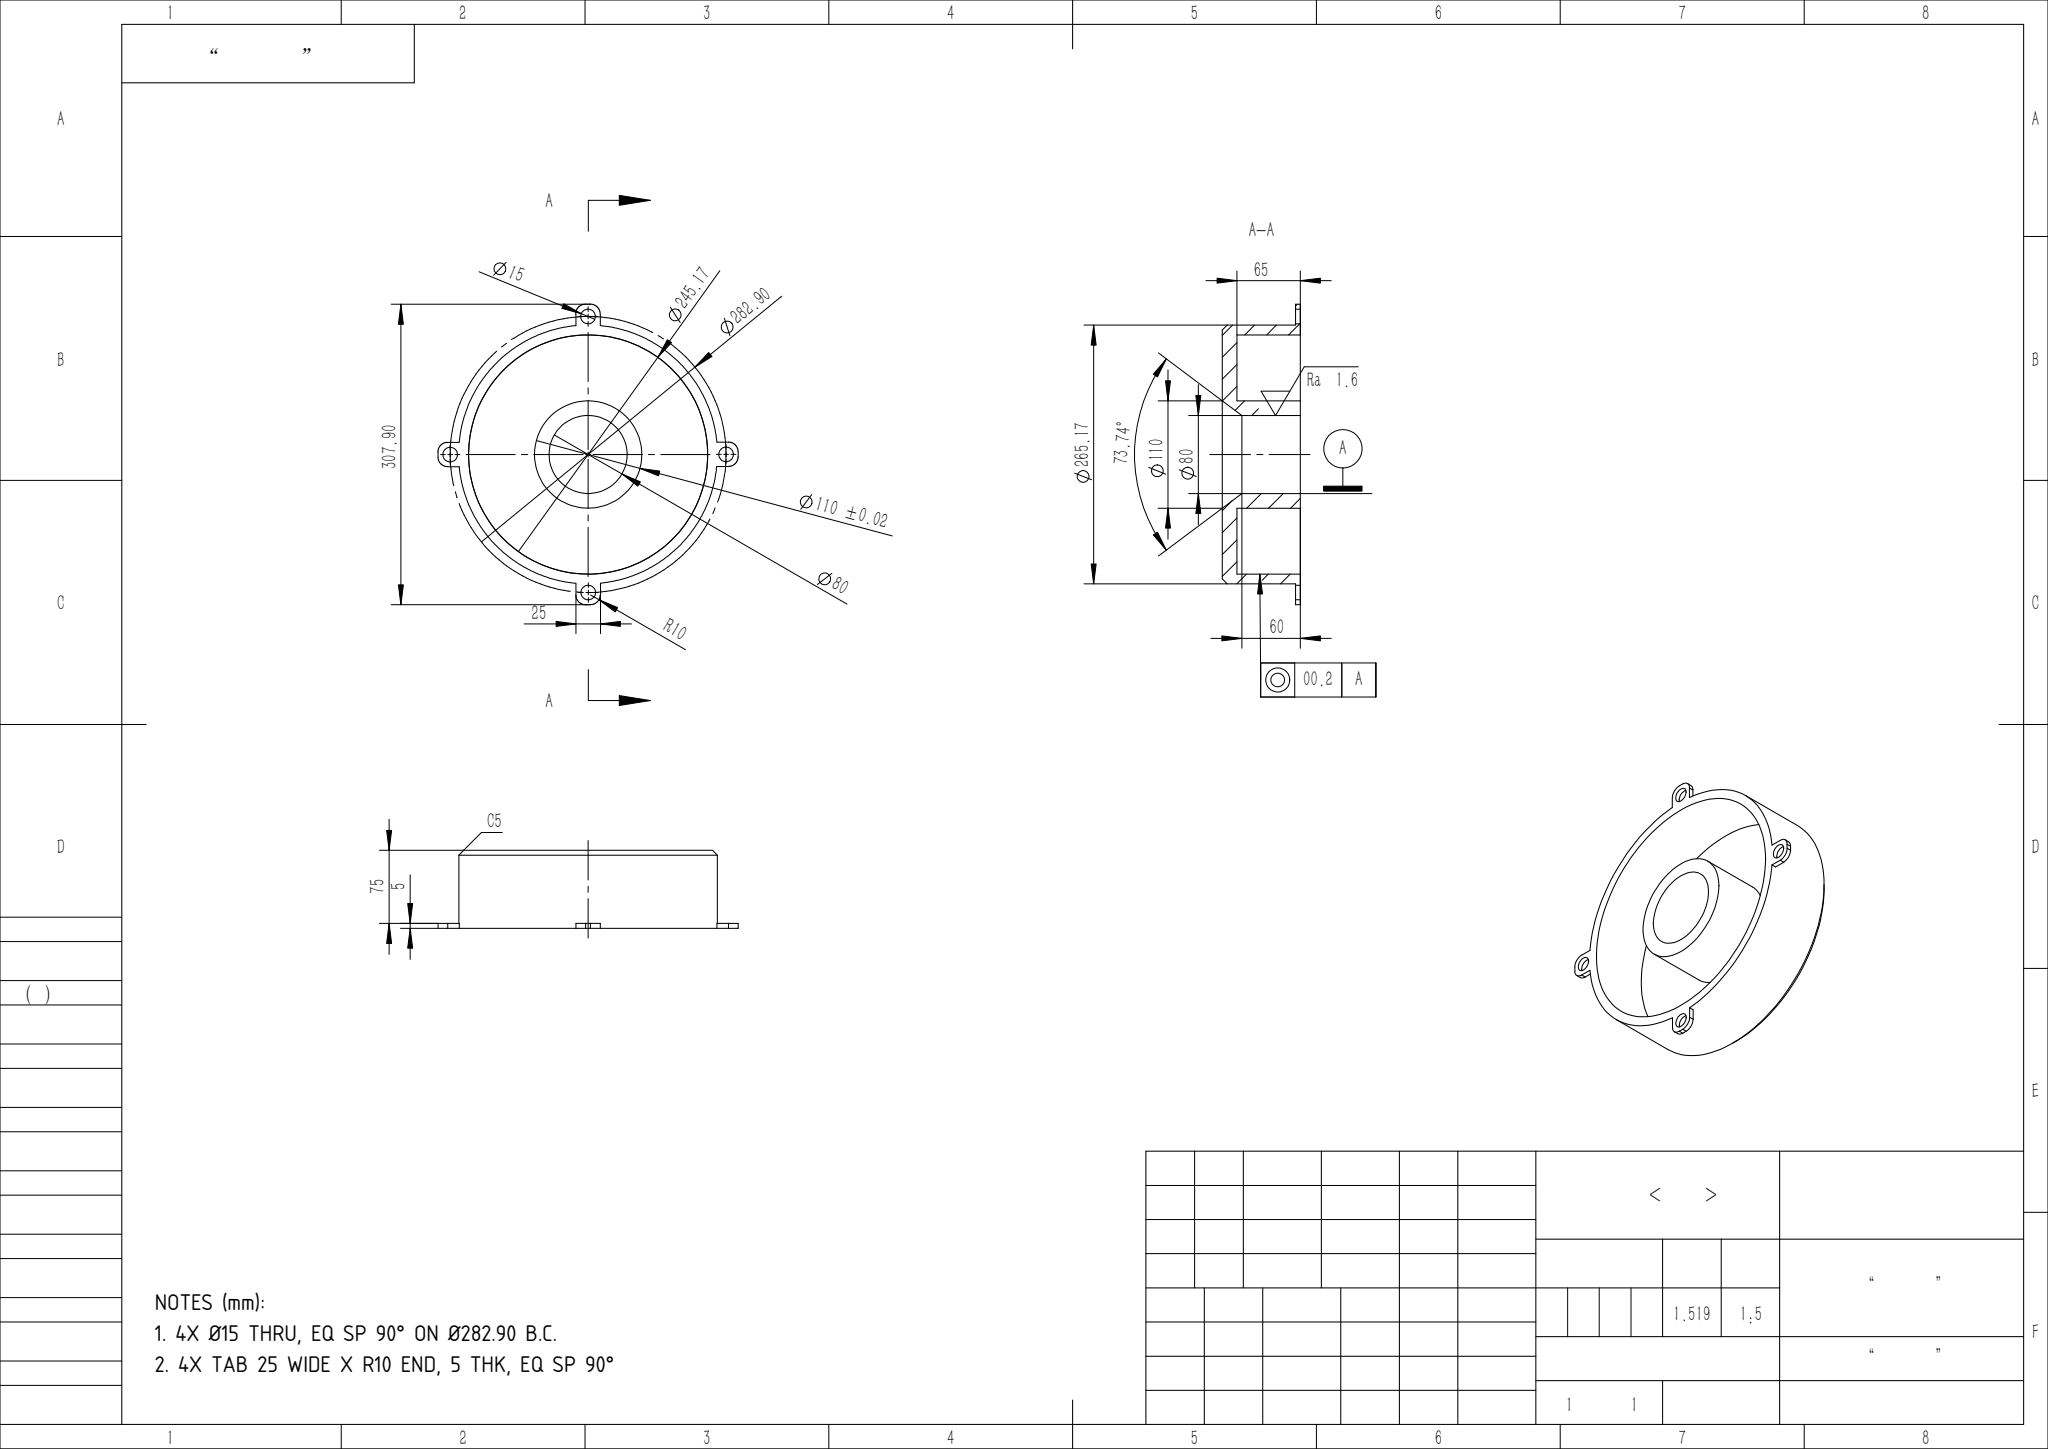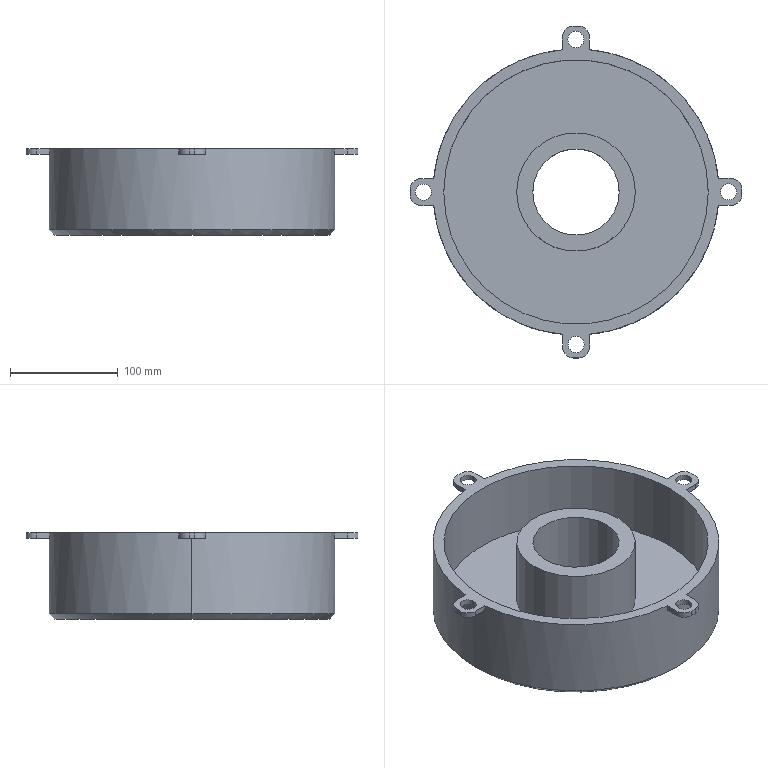Part | SolidWorks | mm | 1 solid | 48 faces | box 307.9 x 307.9 x 80 mm | volume 1518722 mm3 | cylinder 24 | plane 20 | cone 4 | commonest cylinder face diameters 15 x8 20 x8 80 x2 110 x2 245.169 x2 265.169 x2
Drawing notes:
4X Ø15 THRU, EQ SP 90° ON Ø282.90 B.C. | from the solid: Four Ø15 z-cylinders at (12.5,153.85),(153.85,295.4),(154.05,12.5),(295.4,154.05); center (153.95,153.95); radius 141.45 = Ø282.90 B.C., 90° apart
4X TAB 25 WIDE X R10 END, 5 THK, EQ SP 90° | from the solid: Ø20 end cylinders (R10) 5 long at tab ends; planes x/y 141.35 & 166.35 give 25 width; z planes 0 to 5 (15-?) tab thk 5; 4 tabs at 90°
build123d program:
from build123d import *

# Parameters (mm, degrees)
SKETCH1_W                      = 132.584
SKETCH1_H                      = 80
BOSS_EXTRUDE1_REACH            = 327.701
BOSS_EXTRUDE1_END_RADIUS       = 132.584
SKETCH2_W                      = 25
SKETCH2_H                      = 5
BOSS_EXTRUDE2_REACH            = 336.968
BOSS_EXTRUDE2_END_RADIUS       = 132.584
SKETCH3_W                      = 25
SKETCH3_H                      = 5
BOSS_EXTRUDE3_REACH            = 355.419
BOSS_EXTRUDE3_END_RADIUS       = 132.584
SKETCH4_W                      = 5
SKETCH4_H                      = 25
BOSS_EXTRUDE4_REACH            = 355.419
BOSS_EXTRUDE4_END_RADIUS       = 132.584
SKETCH5_W                      = 25
SKETCH5_H                      = 5
HOLE1_D                        = 245.169
HOLE1_DEPTH                    = 65
SKETCH8_W                      = 55
SKETCH8_H                      = 65
F_15_0_15_DIAMETER_HOLE1_D     = 15
F_15_0_15_DIAMETER_HOLE1_DEPTH = 80
M72_CLEARANCE_HOLE1_D          = 80
CHAMFER1_SIZE                  = 15
CHAMFER1_SIZE2                 = 20
CHAMFER2_SIZE                  = 5
FILLET1_R                      = 10


with BuildPart() as part:
    # Sketch1 → Revolve1 (revolve)
    with BuildSketch(Plane(origin=(0, 0, 0), x_dir=(1, 0, 0), z_dir=(0, 1, 0))):
        with Locations((66.292, 40)):
            Rectangle(SKETCH1_W, SKETCH1_H)
    revolve(axis=Axis((0, 0, -80), (0, 0, 1)))

    # Boss-Extrude1: up to this cylinder (the profile starts outside it)
    boss_extrude1_end = Plane(origin=(0, 0, -2.5), z_dir=(0, 0, 1)) * Cylinder(BOSS_EXTRUDE1_END_RADIUS, 921.571, mode=Mode.PRIVATE)
    # Sketch2 → Boss-Extrude1 (add, up to the surface)
    with BuildSketch(Plane.XZ.offset(153.951), mode=Mode.PRIVATE) as boss_extrude1_sk1:
        with Locations((0.1, -2.5)):
            Rectangle(SKETCH2_W, SKETCH2_H)
    boss_extrude1_tool1 = extrude(boss_extrude1_sk1.sketch, amount=-BOSS_EXTRUDE1_REACH, mode=Mode.PRIVATE) - boss_extrude1_end
    add(boss_extrude1_tool1.solids().sort_by_distance((0.1, -153.951, -2.5))[0])

    # Boss-Extrude2: up to this cylinder (the profile starts outside it)
    boss_extrude2_end = Plane(origin=(0, 0, -2.5), z_dir=(0, 0, 1)) * Cylinder(BOSS_EXTRUDE2_END_RADIUS, 940.105, mode=Mode.PRIVATE)
    # Sketch3 → Boss-Extrude2 (add, up to the surface)
    with BuildSketch(Plane(origin=(-153.951, 0, 0), x_dir=(0, -1, 0), z_dir=(-1, 0, 0)), mode=Mode.PRIVATE) as boss_extrude2_sk1:
        with Locations((0.1, -2.5)):
            Rectangle(SKETCH3_W, SKETCH3_H)
    boss_extrude2_tool1 = extrude(boss_extrude2_sk1.sketch, amount=-BOSS_EXTRUDE2_REACH, mode=Mode.PRIVATE) - boss_extrude2_end
    add(boss_extrude2_tool1.solids().sort_by_distance((-153.951, -0.1, -2.5))[0])

    # Boss-Extrude3: up to this cylinder (the profile starts outside it)
    boss_extrude3_end = Plane(origin=(0, 0, -2.5), z_dir=(0, 0, 1)) * Cylinder(BOSS_EXTRUDE3_END_RADIUS, 977.007, mode=Mode.PRIVATE)
    # Sketch4 → Boss-Extrude3 (add, up to the surface)
    with BuildSketch(Plane(origin=(153.951, 0, 0), x_dir=(0, 0, -1), z_dir=(1, 0, 0)), mode=Mode.PRIVATE) as boss_extrude3_sk1:
        with Locations((2.5, 0.1)):
            Rectangle(SKETCH4_W, SKETCH4_H)
    boss_extrude3_tool1 = extrude(boss_extrude3_sk1.sketch, amount=-BOSS_EXTRUDE3_REACH, mode=Mode.PRIVATE) - boss_extrude3_end
    add(boss_extrude3_tool1.solids().sort_by_distance((153.951, 0.1, -2.5))[0])

    # Boss-Extrude4: up to this cylinder (the profile starts outside it)
    boss_extrude4_end = Plane(origin=(0, 0, -2.5), z_dir=(0, 0, 1)) * Cylinder(BOSS_EXTRUDE4_END_RADIUS, 977.007, mode=Mode.PRIVATE)
    # Sketch5 → Boss-Extrude4 (add, up to the surface)
    with BuildSketch(Plane(origin=(0, 153.951, 0), x_dir=(1, 0, 0), z_dir=(0, 1, 0)), mode=Mode.PRIVATE) as boss_extrude4_sk1:
        with Locations((-0.1, 2.5)):
            Rectangle(SKETCH5_W, SKETCH5_H)
    boss_extrude4_tool1 = extrude(boss_extrude4_sk1.sketch, amount=-BOSS_EXTRUDE4_REACH, mode=Mode.PRIVATE) - boss_extrude4_end
    add(boss_extrude4_tool1.solids().sort_by_distance((-0.1, 153.951, -2.5))[0])

    # Hole1
    with Locations(Plane.XY):
        with Locations((0, 0)):
            Hole(HOLE1_D / 2, depth=HOLE1_DEPTH)

    # Sketch8 → Revolve2 (revolve)
    with BuildSketch(Plane(origin=(0, 0, 0), x_dir=(1, 0, 0), z_dir=(0, 1, 0))):
        with Locations((27.5, 32.5)):
            Rectangle(SKETCH8_W, SKETCH8_H)
    revolve(axis=Axis((0, 0, -65), (0, 0, 1)))

    # 15.0 _15_ Diameter Hole1
    with Locations(Plane.XY):
        with Locations((0.1, -141.451), (-141.451, -0.1), (141.451, 0.1), (-0.1, 141.451)):
            Hole(F_15_0_15_DIAMETER_HOLE1_D / 2, depth=F_15_0_15_DIAMETER_HOLE1_DEPTH)

    # M72 Clearance Hole1 (through all)
    with Locations(Plane(origin=(0, 0, -80), x_dir=(-1, 0, 0), z_dir=(0, 0, -1))):
        with Locations((0, 0)):
            Hole(M72_CLEARANCE_HOLE1_D / 2)

    # Chamfer1
    chamfer1_edges = [part.edges().sort_by_distance(p)[0] for p in [
        (-40, 0, -80),
    ]]
    chamfer1_side = [part.faces().sort_by_distance(p)[0] for p in [
        (-128.834, 0, -80),
    ]]
    chamfer(chamfer1_edges, length=CHAMFER1_SIZE, length2=CHAMFER1_SIZE2, reference=chamfer1_side[0])

    # Chamfer2
    chamfer2_edges = [part.edges().sort_by_distance(p)[0] for p in [
        (-132.584, 0, -80),
    ]]
    chamfer(chamfer2_edges, length=CHAMFER2_SIZE)

    # Fillet1
    fillet1_edges = [part.edges().sort_by_distance(p)[0] for p in [
        (12.6, -153.951, -2.5),
        (-12.4, -153.951, -2.5),
        (-153.951, -12.6, -2.5),
        (-153.951, 12.4, -2.5),
        (153.951, 12.6, -2.5),
        (153.951, -12.4, -2.5),
        (-12.6, 153.951, -2.5),
        (12.4, 153.951, -2.5),
    ]]
    fillet(fillet1_edges, radius=FILLET1_R)


solid = part.part